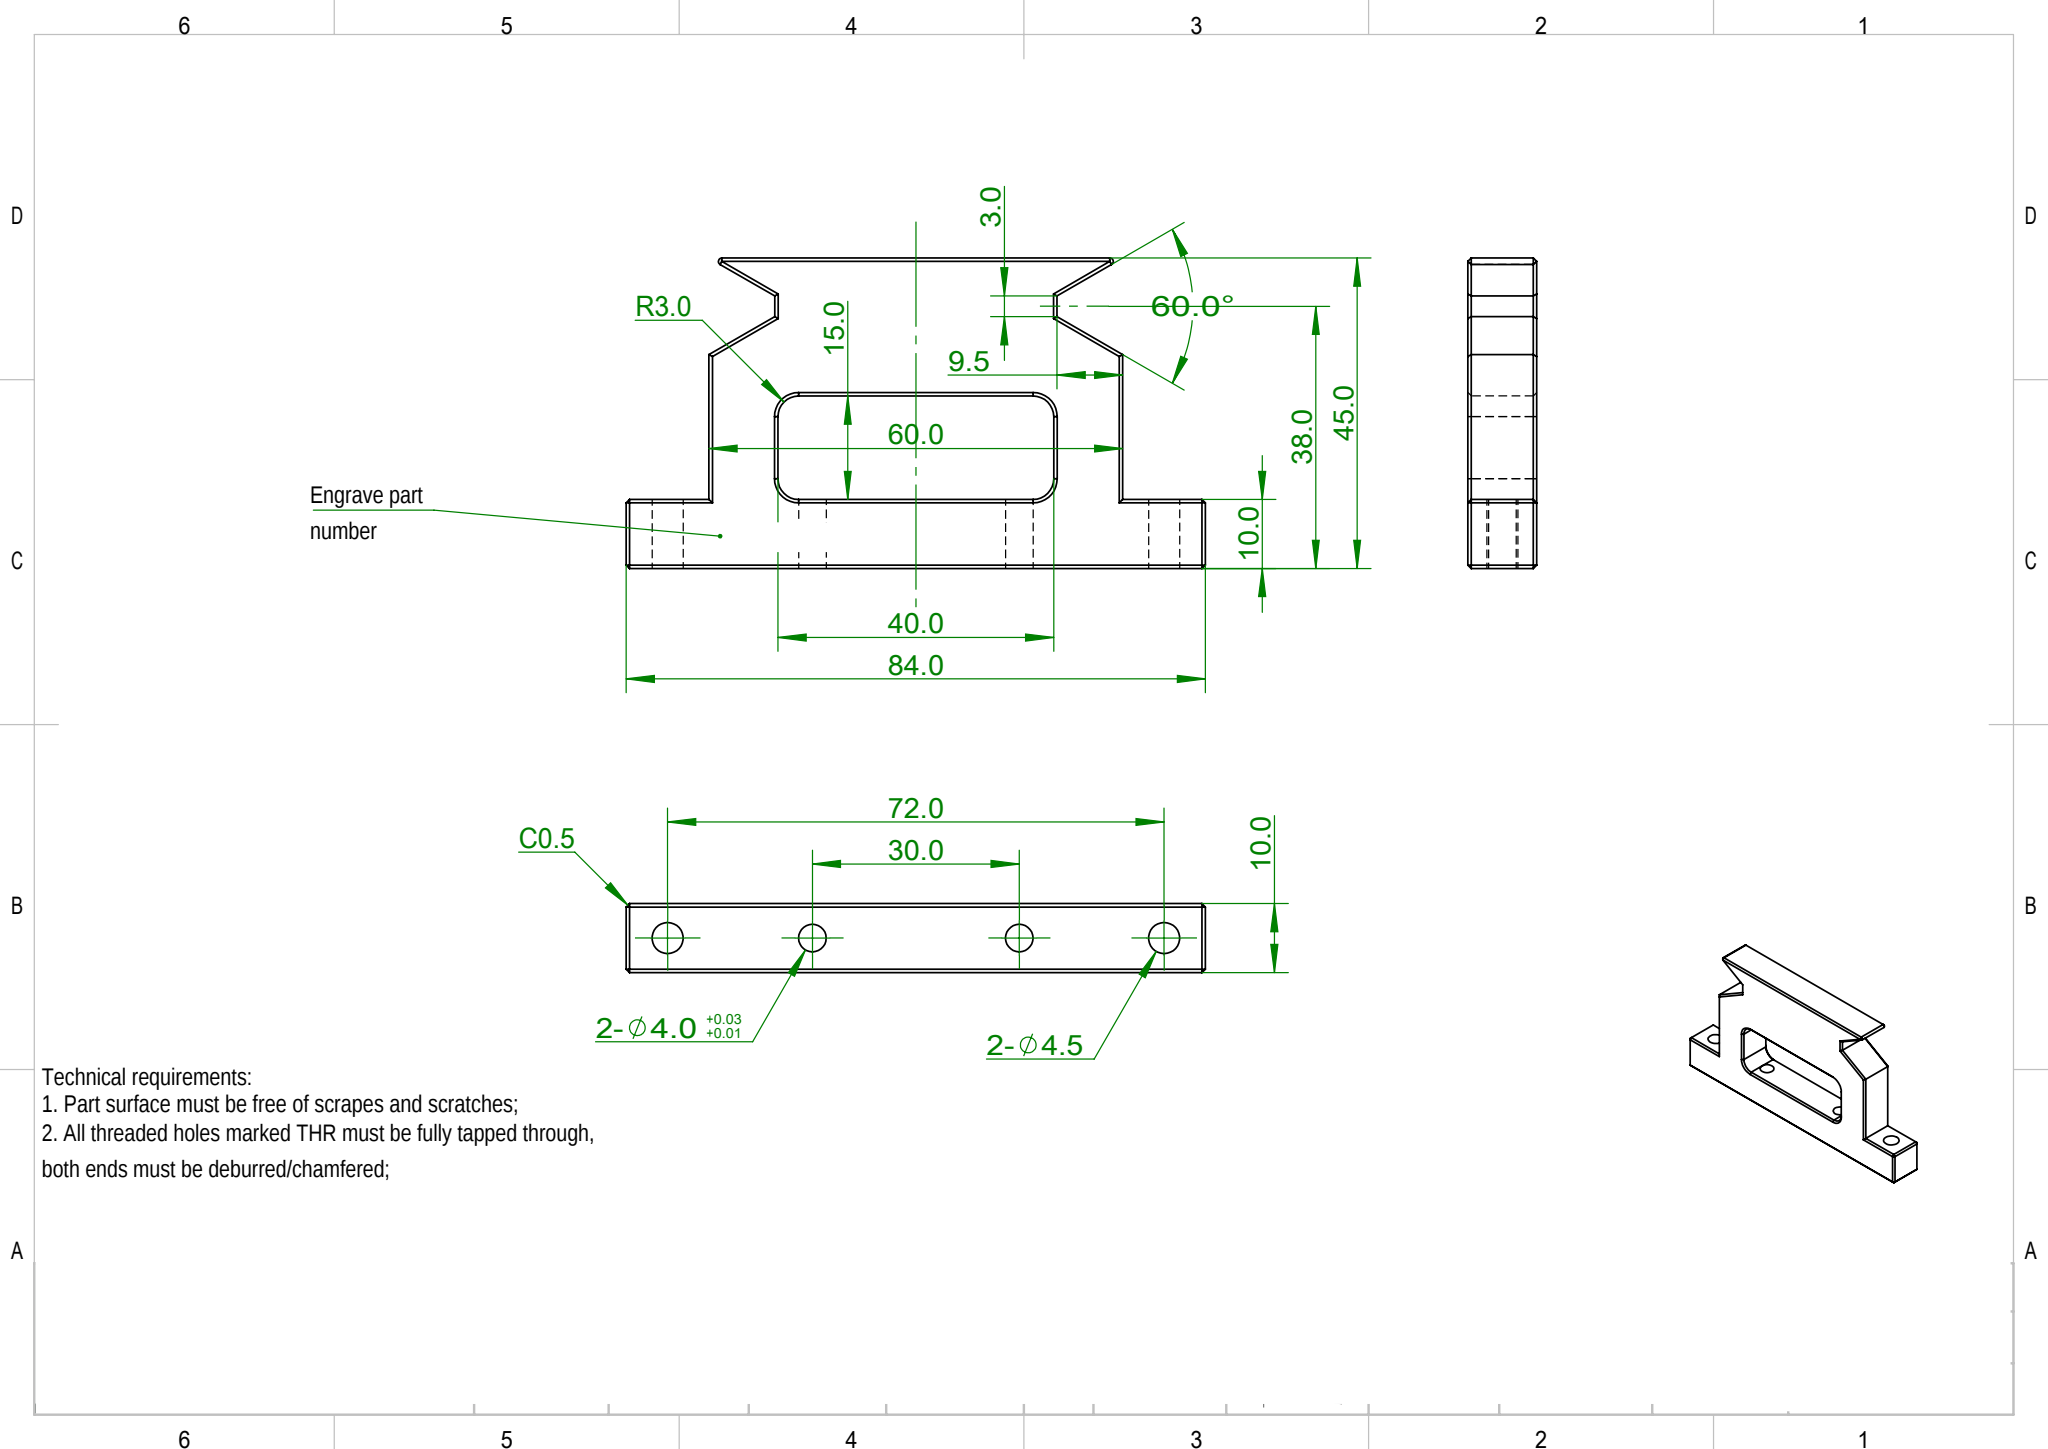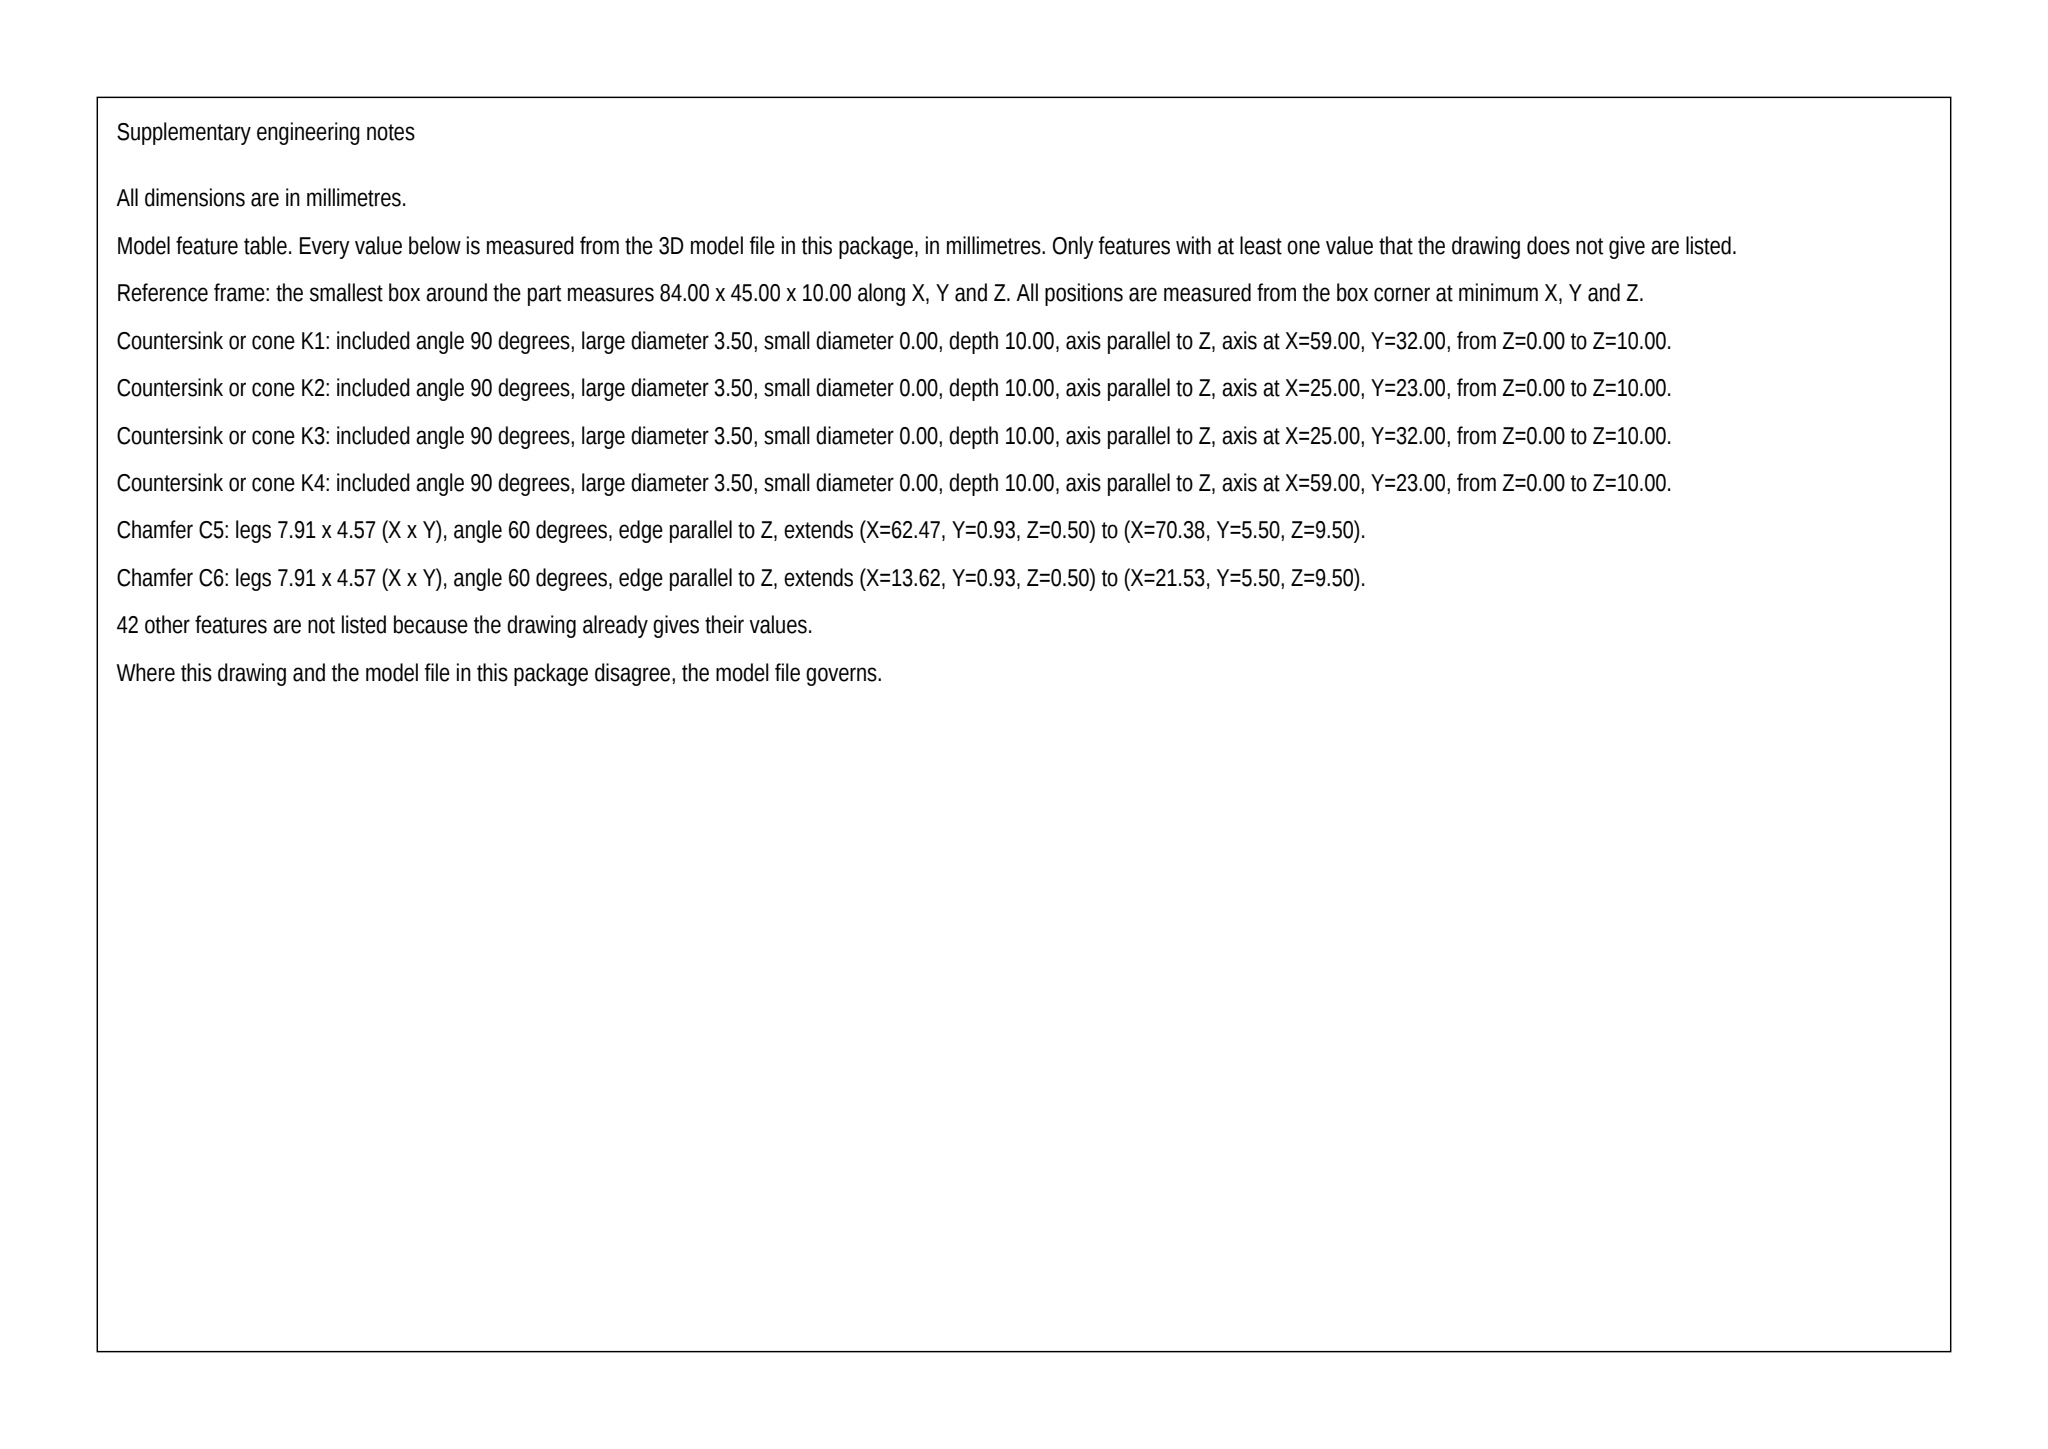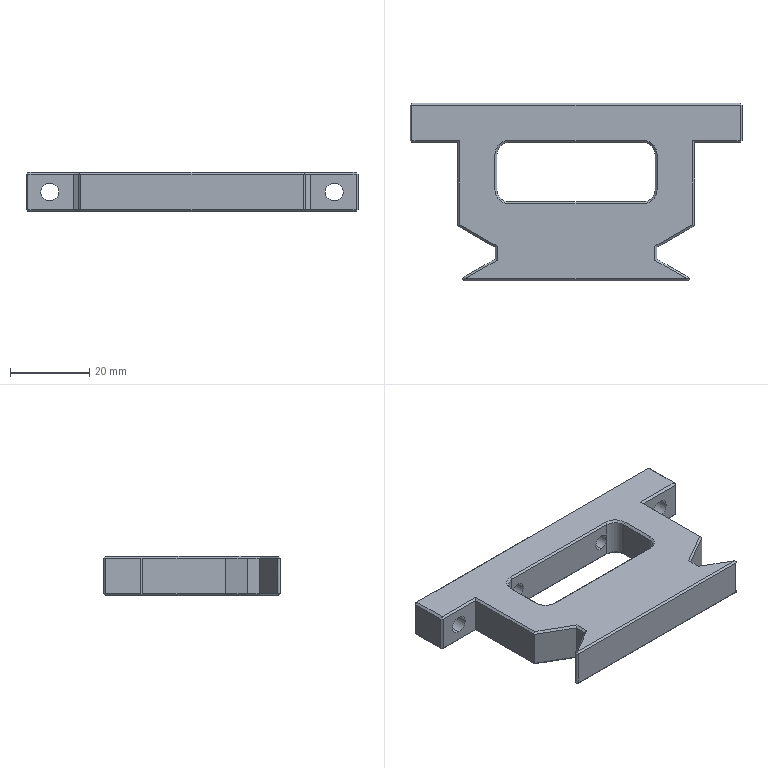Part | SolidWorks | mm | 1 solid | 97 faces | box 84 x 45 x 10 mm | volume 21177 mm3 | plane 68 | cylinder 15 | cone 14 | commonest cylinder face diameters 4 x4 4.5 x4 6 x4 1 x3